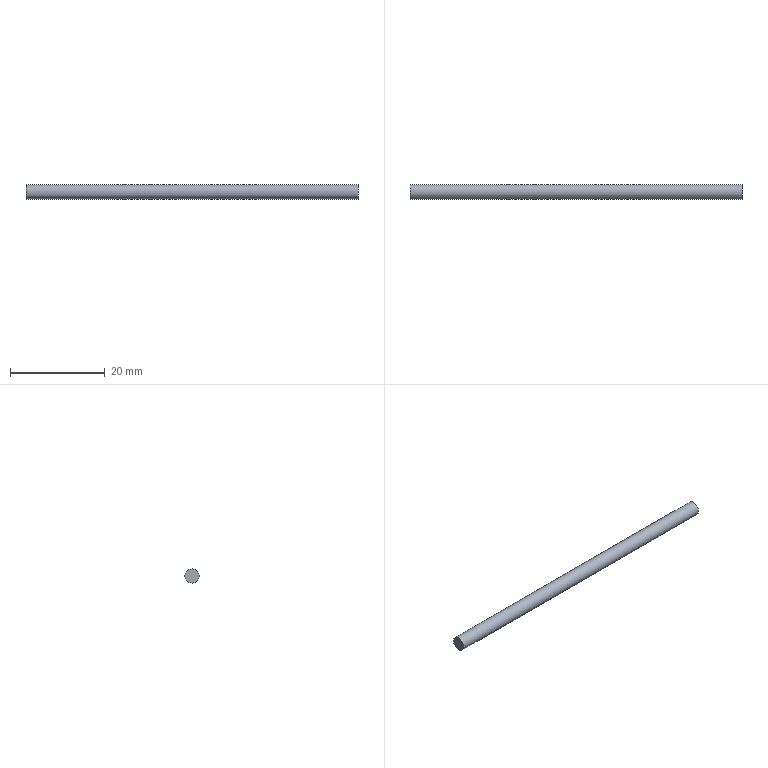Component | NX | PISTON_ROD_2_2 | 1 solid | 3 faces | box 70 x 3 x 3 mm | volume 495 mm3 | plane 2 | cylinder 1 | commonest cylinder face diameters 3 x1
STEP:
#1=CARTESIAN_POINT('',(0.,0.,0.));
#2=DIRECTION('',(0.,0.,1.));
#3=DIRECTION('',(1.,0.,0.));
#4=AXIS2_PLACEMENT_3D('',#1,#2,#3);
#5=CARTESIAN_POINT('',(-99.724,-10.75,42.5));
#6=VERTEX_POINT('',#5);
#7=CARTESIAN_POINT('',(-99.724,-10.75,41.));
#8=DIRECTION('',(1.,0.,0.));
#9=DIRECTION('',(0.,0.,1.));
#10=AXIS2_PLACEMENT_3D('',#7,#8,#9);
#11=CIRCLE('',#10,1.5);
#12=CARTESIAN_POINT('',(-99.724,-10.75,41.));
#13=DIRECTION('',(-1.,0.,0.));
#14=DIRECTION('',(0.,0.,1.));
#15=AXIS2_PLACEMENT_3D('',#12,#13,#14);
#16=PLANE('',#15);
#17=CARTESIAN_POINT('',(1.5,0.));
#18=CARTESIAN_POINT('',(1.5,-2.598));
#19=CARTESIAN_POINT('',(-0.75,-1.299));
#20=CARTESIAN_POINT('',(-3.,-0.));
#21=CARTESIAN_POINT('',(-0.75,1.299));
#22=CARTESIAN_POINT('',(1.5,2.598));
#23=CARTESIAN_POINT('',(1.5,0.));
#24=(BOUNDED_CURVE()B_SPLINE_CURVE(2,(#17,#18,#19,#20,#21,#22,#23),.UNSPECIFIED.,.T.,.F.)B_SPLINE_CURVE_WITH_KNOTS((1,2,2,2,2,1),(-2.094,0.,2.094,4.189,6.283,8.378),.UNSPECIFIED.)CURVE()GEOMETRIC_REPRESENTATION_ITEM()RATIONAL_B_SPLINE_CURVE((1.,0.5,1.,0.5,1.,0.5,1.))REPRESENTATION_ITEM(''));
#25=(GEOMETRIC_REPRESENTATION_CONTEXT(2)PARAMETRIC_REPRESENTATION_CONTEXT()REPRESENTATION_CONTEXT('',''));
#26=DEFINITIONAL_REPRESENTATION('',(#24),#25);
#27=PCURVE('',#16,#26);
#28=CARTESIAN_POINT('',(-29.724,-10.75,41.));
#29=DIRECTION('',(-1.,0.,0.));
#30=DIRECTION('',(0.,0.,1.));
#31=AXIS2_PLACEMENT_3D('',#28,#29,#30);
#32=CYLINDRICAL_SURFACE('',#31,1.5);
#33=CARTESIAN_POINT('',(6.283,70.));
#34=DIRECTION('',(-1.,0.));
#35=VECTOR('',#34,1.);
#36=LINE('',#33,#35);
#37=(GEOMETRIC_REPRESENTATION_CONTEXT(2)PARAMETRIC_REPRESENTATION_CONTEXT()REPRESENTATION_CONTEXT('',''));
#38=DEFINITIONAL_REPRESENTATION('',(#36),#37);
#39=PCURVE('',#32,#38);
#40=SURFACE_CURVE('',#11,(#27,#39),.PCURVE_S1.);
#41=EDGE_CURVE('',#6,#6,#40,.T.);
#42=ORIENTED_EDGE('',*,*,#41,.F.);
#43=EDGE_LOOP('',(#42));
#44=FACE_BOUND('',#43,.T.);
#45=ADVANCED_FACE('',(#44),#16,.T.);
#46=CARTESIAN_POINT('',(-29.724,-10.75,42.5));
#47=VERTEX_POINT('',#46);
#48=CARTESIAN_POINT('',(-29.724,-10.75,41.));
#49=DIRECTION('',(-1.,0.,0.));
#50=DIRECTION('',(0.,0.,1.));
#51=AXIS2_PLACEMENT_3D('',#48,#49,#50);
#52=CIRCLE('',#51,1.5);
#53=CARTESIAN_POINT('',(-29.724,-10.75,41.));
#54=DIRECTION('',(1.,0.,0.));
#55=DIRECTION('',(0.,0.,-1.));
#56=AXIS2_PLACEMENT_3D('',#53,#54,#55);
#57=PLANE('',#56);
#58=CARTESIAN_POINT('',(-1.5,0.));
#59=CARTESIAN_POINT('',(-1.5,2.598));
#60=CARTESIAN_POINT('',(0.75,1.299));
#61=CARTESIAN_POINT('',(3.,0.));
#62=CARTESIAN_POINT('',(0.75,-1.299));
#63=CARTESIAN_POINT('',(-1.5,-2.598));
#64=CARTESIAN_POINT('',(-1.5,0.));
#65=(BOUNDED_CURVE()B_SPLINE_CURVE(2,(#58,#59,#60,#61,#62,#63,#64),.UNSPECIFIED.,.T.,.F.)B_SPLINE_CURVE_WITH_KNOTS((1,2,2,2,2,1),(-2.094,0.,2.094,4.189,6.283,8.378),.UNSPECIFIED.)CURVE()GEOMETRIC_REPRESENTATION_ITEM()RATIONAL_B_SPLINE_CURVE((1.,0.5,1.,0.5,1.,0.5,1.))REPRESENTATION_ITEM(''));
#66=(GEOMETRIC_REPRESENTATION_CONTEXT(2)PARAMETRIC_REPRESENTATION_CONTEXT()REPRESENTATION_CONTEXT('',''));
#67=DEFINITIONAL_REPRESENTATION('',(#65),#66);
#68=PCURVE('',#57,#67);
#69=CARTESIAN_POINT('',(0.,0.));
#70=DIRECTION('',(1.,0.));
#71=VECTOR('',#70,1.);
#72=LINE('',#69,#71);
#73=(GEOMETRIC_REPRESENTATION_CONTEXT(2)PARAMETRIC_REPRESENTATION_CONTEXT()REPRESENTATION_CONTEXT('',''));
#74=DEFINITIONAL_REPRESENTATION('',(#72),#73);
#75=PCURVE('',#32,#74);
#76=SURFACE_CURVE('',#52,(#68,#75),.PCURVE_S1.);
#77=EDGE_CURVE('',#47,#47,#76,.T.);
#78=ORIENTED_EDGE('',*,*,#77,.F.);
#79=EDGE_LOOP('',(#78));
#80=FACE_BOUND('',#79,.T.);
#81=ADVANCED_FACE('',(#80),#57,.T.);
#82=ORIENTED_EDGE('',*,*,#41,.T.);
#83=CARTESIAN_POINT('',(-29.724,-10.75,42.5));
#84=CARTESIAN_POINT('',(-99.724,-10.75,42.5));
#85=B_SPLINE_CURVE_WITH_KNOTS('',1,(#83,#84),.UNSPECIFIED.,.F.,.F.,(2,2),(0.,70.),.PIECEWISE_BEZIER_KNOTS.);
#86=CARTESIAN_POINT('',(0.,0.));
#87=DIRECTION('',(0.,1.));
#88=VECTOR('',#87,1.);
#89=LINE('',#86,#88);
#90=(GEOMETRIC_REPRESENTATION_CONTEXT(2)PARAMETRIC_REPRESENTATION_CONTEXT()REPRESENTATION_CONTEXT('',''));
#91=DEFINITIONAL_REPRESENTATION('',(#89),#90);
#92=PCURVE('',#32,#91);
#93=CARTESIAN_POINT('',(6.283,0.));
#94=DIRECTION('',(0.,1.));
#95=VECTOR('',#94,1.);
#96=LINE('',#93,#95);
#97=(GEOMETRIC_REPRESENTATION_CONTEXT(2)PARAMETRIC_REPRESENTATION_CONTEXT()REPRESENTATION_CONTEXT('',''));
#98=DEFINITIONAL_REPRESENTATION('',(#96),#97);
#99=PCURVE('',#32,#98);
#100=SEAM_CURVE('',#85,(#92,#99),.PCURVE_S1.);
#101=EDGE_CURVE('',#47,#6,#100,.T.);
#102=ORIENTED_EDGE('',*,*,#101,.F.);
#103=ORIENTED_EDGE('',*,*,#77,.T.);
#104=ORIENTED_EDGE('',*,*,#101,.T.);
#105=EDGE_LOOP('',(#82,#102,#103,#104));
#106=FACE_BOUND('',#105,.T.);
#107=ADVANCED_FACE('',(#106),#32,.T.);
#108=CLOSED_SHELL('',(#45,#81,#107));
#109=MANIFOLD_SOLID_BREP('',#108);
#110=(LENGTH_UNIT()NAMED_UNIT(*)SI_UNIT(.MILLI.,.METRE.));
#111=UNCERTAINTY_MEASURE_WITH_UNIT(LENGTH_MEASURE(0.00001),#110,'','');
#112=(NAMED_UNIT(*)PLANE_ANGLE_UNIT()SI_UNIT($,.RADIAN.));
#113=(NAMED_UNIT(*)SI_UNIT($,.STERADIAN.)SOLID_ANGLE_UNIT());
#114=(GEOMETRIC_REPRESENTATION_CONTEXT(3)GLOBAL_UNCERTAINTY_ASSIGNED_CONTEXT((#111))GLOBAL_UNIT_ASSIGNED_CONTEXT((#110,#112,#113))REPRESENTATION_CONTEXT('',''));
#115=ADVANCED_BREP_SHAPE_REPRESENTATION('',(#4,#109),#114);